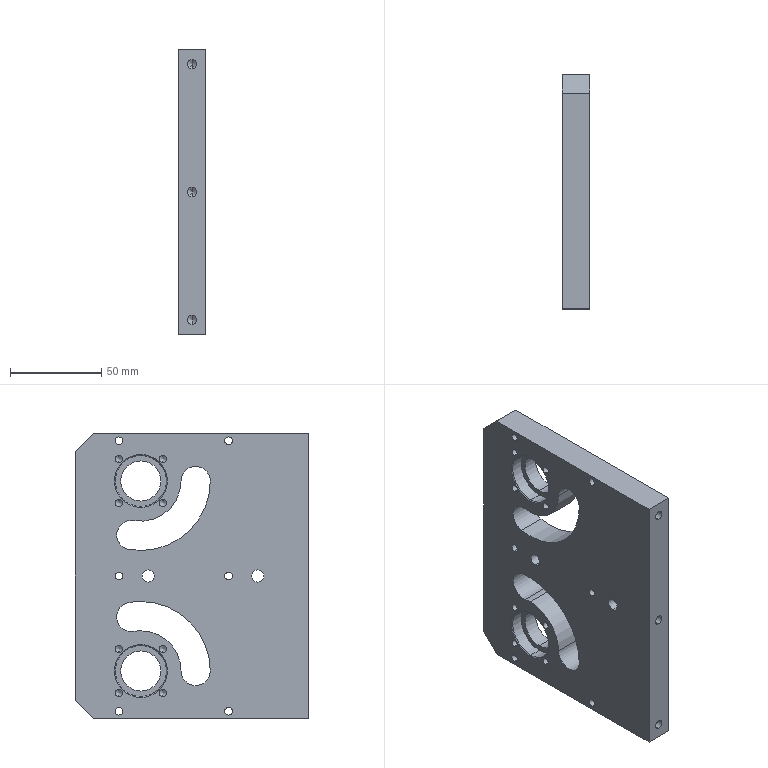Component | SolidWorks | ClampingAssembly-1_A70-1 | 1 solid | 116 faces | box 15 x 128 x 156 mm | volume 246351 mm3 | cylinder 70 | cone 34 | plane 12 | commonest cylinder face diameters 4.2 x20 4 x16 5 x6 16 x6 28 x4 11 x4 6.6 x4 22 x4 | material S136
build123d program:
from build123d import *

# Parameters (mm, degrees)
SKETCH1_W                                          = 156
SKETCH1_H                                          = 128
BOSS_EXTRUDE1_DEPTH                                = 7.5
SKETCH2_R                                          = 11
CUT_EXTRUDE1_DEPTH                                 = 103.005
SKETCH3_R                                          = 14
CUT_EXTRUDE2_DEPTH                                 = 7
CHAMFER1_SIZE                                      = 0.5
M4_TAPPED_HOLE1_AT_2_COUNT                         = 2
M4_TAPPED_HOLE1_AT_2_PITCH                         = 34
M4_TAPPED_HOLE1_AT_3_COUNT                         = 2
M4_TAPPED_HOLE1_AT_3_PITCH                         = 24.042
M4_TAPPED_HOLE1_AT_4_COUNT                         = 2
M4_TAPPED_HOLE1_AT_4_PITCH                         = 24.042
CUT_EXTRUDE3_DEPTH                                 = 103.005
CHAMFER2_SIZE                                      = 10
M5_TAPPED_HOLE1_D                                  = 4.2
HOLE_SIZE_ACCORDING_TO_TYPE_1_OF_HEXAG_D           = 6.6
HOLE_SIZE_ACCORDING_TO_TYPE_1_OF_HEXAG_CBORE_D     = 11
HOLE_SIZE_ACCORDING_TO_TYPE_1_OF_HEXAG_CBORE_DEPTH = 6.8
CHAMFER1_OF_MIRROR1_SIZE                           = 0.5
M5_TAPPED_HOLE2_D                                  = 4.2
M5_TAPPED_HOLE2_DEPTH                              = 12.4
M5_TAPPED_HOLE2_TIP                                = 1.262
M6_TAPPED_HOLE1_D                                  = 5
M6_TAPPED_HOLE1_DEPTH                              = 15
M6_TAPPED_HOLE1_TIP                                = 1.502


with BuildPart() as part:
    # Sketch1 → Boss-Extrude1 (new, symmetric)
    with BuildSketch(Plane(origin=(0, 0, 0), x_dir=(0, 0, -1), z_dir=(1, 0, 0))):
        Rectangle(SKETCH1_W, SKETCH1_H)
    extrude(amount=BOSS_EXTRUDE1_DEPTH, both=True)

    # Sketch2 → Cut-Extrude1 (cut, through all)
    with BuildSketch(Plane(origin=(7.5, 0, 0), x_dir=(0, 0, -1), z_dir=(1, 0, 0))):
        with Locations((52, 28)):
            Circle(SKETCH2_R)
    cut_extrude1 = extrude(amount=-CUT_EXTRUDE1_DEPTH, mode=Mode.SUBTRACT)

    # Sketch3 → Cut-Extrude2 (cut)
    with BuildSketch(Plane.ZY.offset(7.5)):
        with Locations((-52, 28)):
            Circle(SKETCH3_R)
    cut_extrude2 = extrude(amount=-CUT_EXTRUDE2_DEPTH, mode=Mode.SUBTRACT)

    # Chamfer1
    chamfer1_edges = [part.edges().sort_by_distance(p)[0] for p in [
        (-7.5, 28, -66),
    ]]
    chamfer(chamfer1_edges, length=CHAMFER1_SIZE)

    # Sketch5 → M4 Tapped Hole1 (revolve, cut)
    with BuildSketch(Plane(origin=(-7.5, 15.979, -64.021), x_dir=(0, 0, 1), z_dir=(0, 1, 0))):
        Polygon((0, 0), (0, 11.302), (2, 10.1), (2, 0), align=None)
    m4_tapped_hole1 = revolve(axis=Axis((-13.85, 15.979, -64.021), (1, 0, 0)), mode=Mode.SUBTRACT)

    # M4 Tapped Hole1 at 2: M4 Tapped Hole1 ×2
    with Locations(*[Vector(0, 0.7071, 0.7071) * (i * M4_TAPPED_HOLE1_AT_2_PITCH) for i in range(1, M4_TAPPED_HOLE1_AT_2_COUNT)]):
        add(m4_tapped_hole1, mode=Mode.SUBTRACT)

    # M4 Tapped Hole1 at 3: M4 Tapped Hole1 ×2
    with Locations(*[(0, 0, i * M4_TAPPED_HOLE1_AT_3_PITCH) for i in range(1, M4_TAPPED_HOLE1_AT_3_COUNT)]):
        add(m4_tapped_hole1, mode=Mode.SUBTRACT)

    # M4 Tapped Hole1 at 4: M4 Tapped Hole1 ×2
    with Locations(*[(0, i * M4_TAPPED_HOLE1_AT_4_PITCH, 0) for i in range(1, M4_TAPPED_HOLE1_AT_4_COUNT)]):
        add(m4_tapped_hole1, mode=Mode.SUBTRACT)

    # Sketch6 → Cut-Extrude3 (cut, through all)
    with BuildSketch(Plane.ZY.offset(7.5)):
        with BuildLine():
            ThreePointArc((-52, -10), (-22.89, 3.574), (-14.577, 34.599))
            ThreePointArc((-14.577, 34.599), (-23.845, 41.088), (-30.334, 31.82))
            ThreePointArc((-30.334, 31.82), (-35.147, 13.859), (-52, 6))
            ThreePointArc((-52, 6), (-60, -2), (-52, -10))
        make_face()
    cut_extrude3 = extrude(amount=-CUT_EXTRUDE3_DEPTH, mode=Mode.SUBTRACT)

    # Chamfer2
    chamfer2_edges = [part.edges().sort_by_distance(p)[0] for p in [
        (0, 64, 78),
        (0, 64, -78),
    ]]
    chamfer(chamfer2_edges, length=CHAMFER2_SIZE)

    # M5 Tapped Hole1 (through all)
    with Locations(Plane(origin=(7.5, 0, 0), x_dir=(0, 0, -1), z_dir=(1, 0, 0))):
        with Locations((0, 40), (0, -20), (74, -20), (74, 40), (-74, -20), (-74, 40)):
            Hole(M5_TAPPED_HOLE1_D / 2)

    # Hole Size _According to_ Type 1 of Hexag (through all)
    with Locations(Plane(origin=(7.5, 0, 0), x_dir=(0, 0, -1), z_dir=(1, 0, 0))):
        with Locations((0, 24), (0, -36)):
            CounterBoreHole(HOLE_SIZE_ACCORDING_TO_TYPE_1_OF_HEXAG_D / 2, HOLE_SIZE_ACCORDING_TO_TYPE_1_OF_HEXAG_CBORE_D / 2, HOLE_SIZE_ACCORDING_TO_TYPE_1_OF_HEXAG_CBORE_DEPTH)

    # Mirror1: Cut-Extrude1, Cut-Extrude2, M4 Tapped Hole1, Cut-Extrude3 across plane
    add(cut_extrude1.mirror(Plane.XY), mode=Mode.SUBTRACT)
    add(cut_extrude2.mirror(Plane.XY), mode=Mode.SUBTRACT)
    add(m4_tapped_hole1.mirror(Plane.XY), mode=Mode.SUBTRACT)
    add(cut_extrude3.mirror(Plane.XY), mode=Mode.SUBTRACT)

    # Mirror1 copy 1 sketch → Mirror1 copy 1 (revolve, cut)
    with BuildSketch(Plane(origin=(-7.5, 40.021, 39.979), x_dir=(0, 0, -1), z_dir=(0, 1, 0))):
        Polygon((0, 0), (0, -11.302), (2, -10.1), (2, 0), align=None)
    revolve(axis=Axis((-13.85, 40.021, 39.979), (-1, 0, 0)), mode=Mode.SUBTRACT)

    # Mirror1 copy 2 sketch → Mirror1 copy 2 (revolve, cut)
    with BuildSketch(Plane(origin=(-7.5, 15.979, 39.979), x_dir=(0, 0, -1), z_dir=(0, 1, 0))):
        Polygon((0, 0), (0, -11.302), (2, -10.1), (2, 0), align=None)
    revolve(axis=Axis((-13.85, 15.979, 39.979), (-1, 0, 0)), mode=Mode.SUBTRACT)

    # Mirror1 copy 3 sketch → Mirror1 copy 3 (revolve, cut)
    with BuildSketch(Plane(origin=(-7.5, 40.021, 64.021), x_dir=(0, 0, -1), z_dir=(0, 1, 0))):
        Polygon((0, 0), (0, -11.302), (2, -10.1), (2, 0), align=None)
    revolve(axis=Axis((-13.85, 40.021, 64.021), (-1, 0, 0)), mode=Mode.SUBTRACT)

    # Chamfer1 of Mirror1
    chamfer1_of_mirror1_edges = [part.edges().sort_by_distance(p)[0] for p in [
        (-7.5, 28, 66),
    ]]
    chamfer(chamfer1_of_mirror1_edges, length=CHAMFER1_OF_MIRROR1_SIZE)

    # M5 Tapped Hole2
    with Locations(Plane(origin=(0, 64, 0), x_dir=(1, 0, 0), z_dir=(0, 1, 0))):
        with Locations((-1.5, 46), (-1.5, 28), (-1.5, -28), (-1.5, -46)):
            Hole(M5_TAPPED_HOLE2_D / 2, depth=M5_TAPPED_HOLE2_DEPTH)
            with Locations((0, 0, -(M5_TAPPED_HOLE2_DEPTH + M5_TAPPED_HOLE2_TIP / 2))):  # 118° drill point
                Cone(0, M5_TAPPED_HOLE2_D / 2, M5_TAPPED_HOLE2_TIP, mode=Mode.SUBTRACT)

    # M6 Tapped Hole1
    with Locations(Plane(origin=(0, -64, 0), x_dir=(-1, 0, 0), z_dir=(0, -1, 0))):
        with Locations((0, 0), (0, -70), (0, 70)):
            Hole(M6_TAPPED_HOLE1_D / 2, depth=M6_TAPPED_HOLE1_DEPTH)
            with Locations((0, 0, -(M6_TAPPED_HOLE1_DEPTH + M6_TAPPED_HOLE1_TIP / 2))):  # 118° drill point
                Cone(0, M6_TAPPED_HOLE1_D / 2, M6_TAPPED_HOLE1_TIP, mode=Mode.SUBTRACT)


solid = part.part

# Placed as in the assembly
solid = solid.moved(Location((-22.051, 38.036, -0.5), (0, 0, 0)))